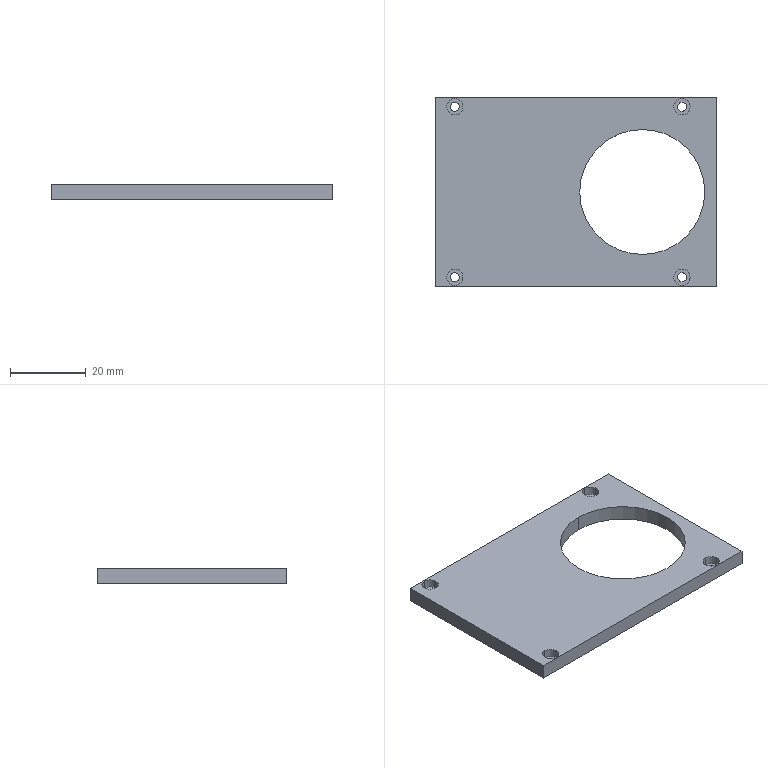CAM job | Mastercam | mm | 14 operations | part box 74 x 50 x 4
1. Facing | 24 - 80 平铣刀
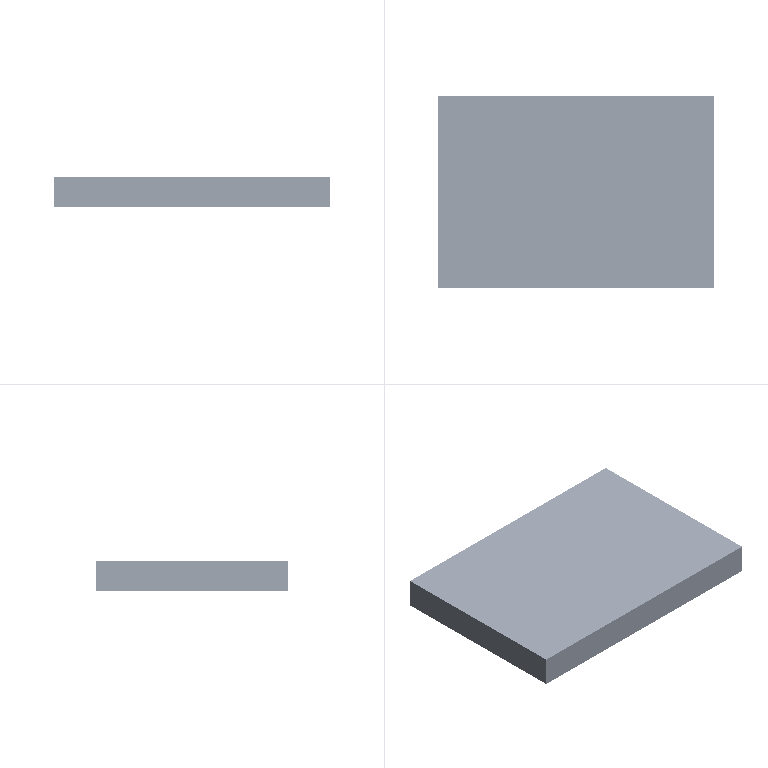2. 3D High Speed (Dynamic OptiRough) | 8 - 8C
3. Drill/Counterbore | 1 - 6 倒角刀
4. Peck Drill | 7 - 2.4 钻头
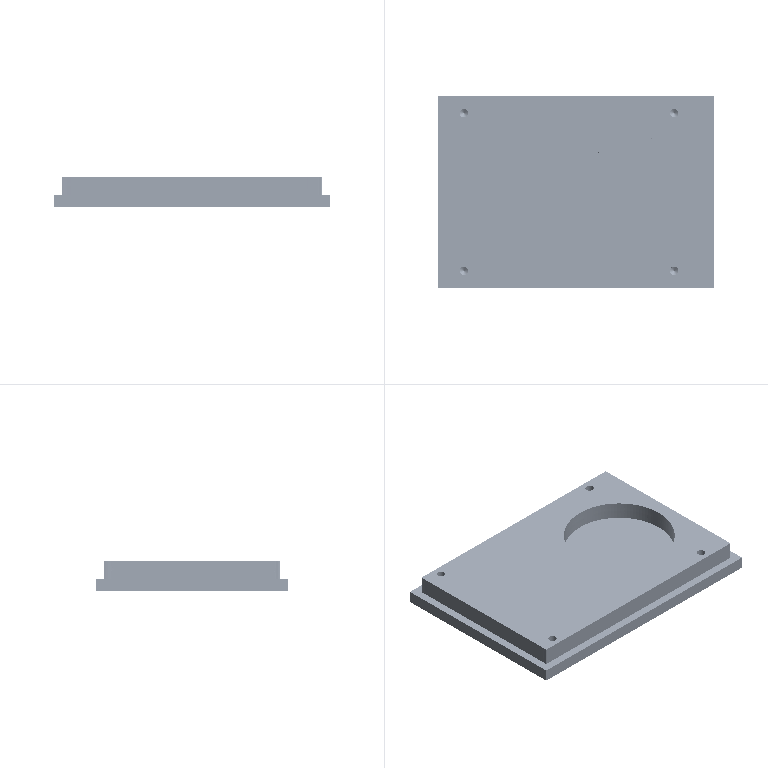5. Contour (Ramp) | 12 - 3C
6. Contour (2D) | 13 - 3J
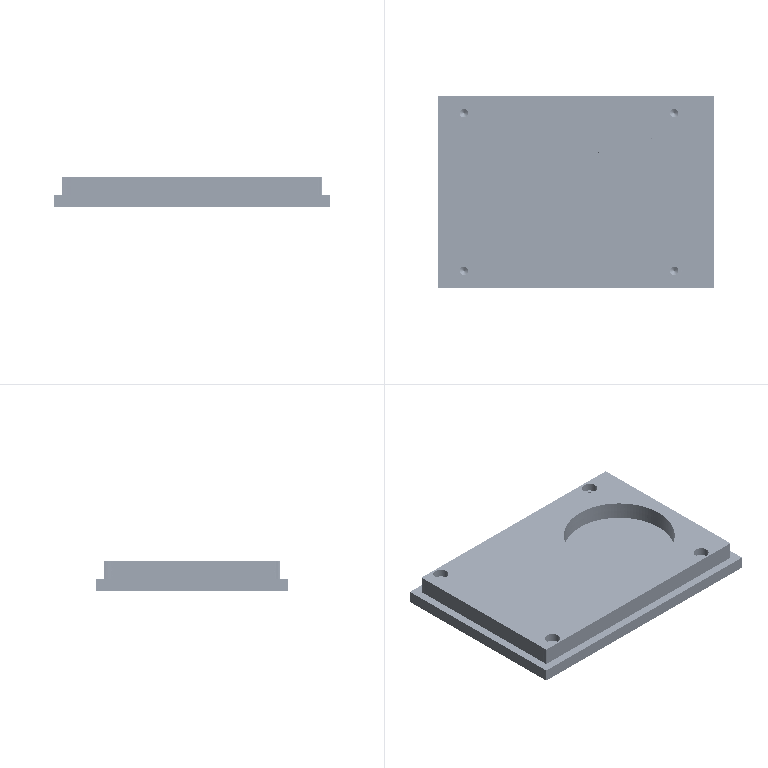7. Contour (2D) | 9 - 8J
8. Contour (2D chamfer) | 1 - 6 倒角刀
9. Facing | 24 - 80 平铣刀
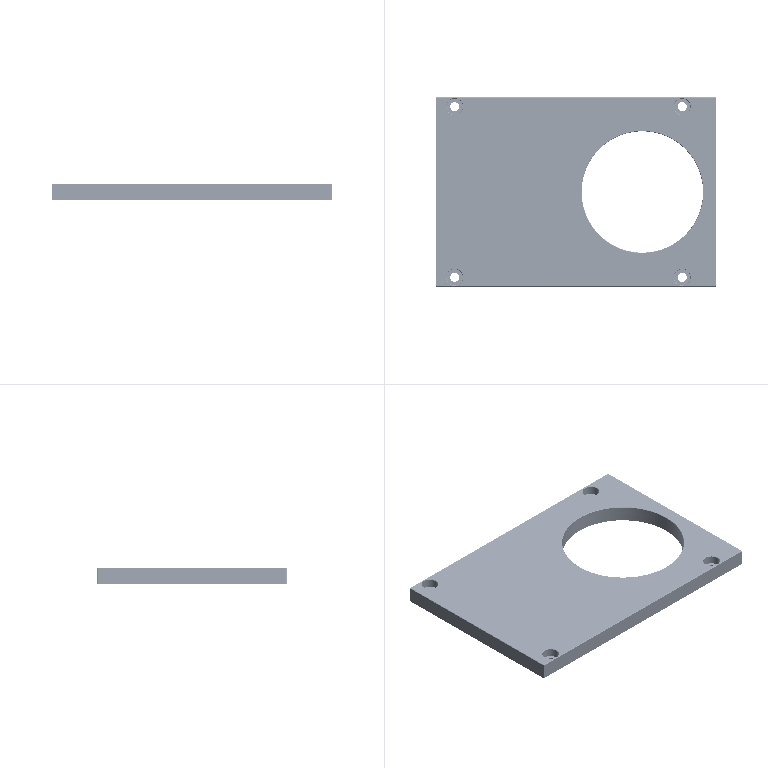10. Facing | 24 - 80 平铣刀
11. Contour (2D chamfer) | 1 - 6 倒角刀
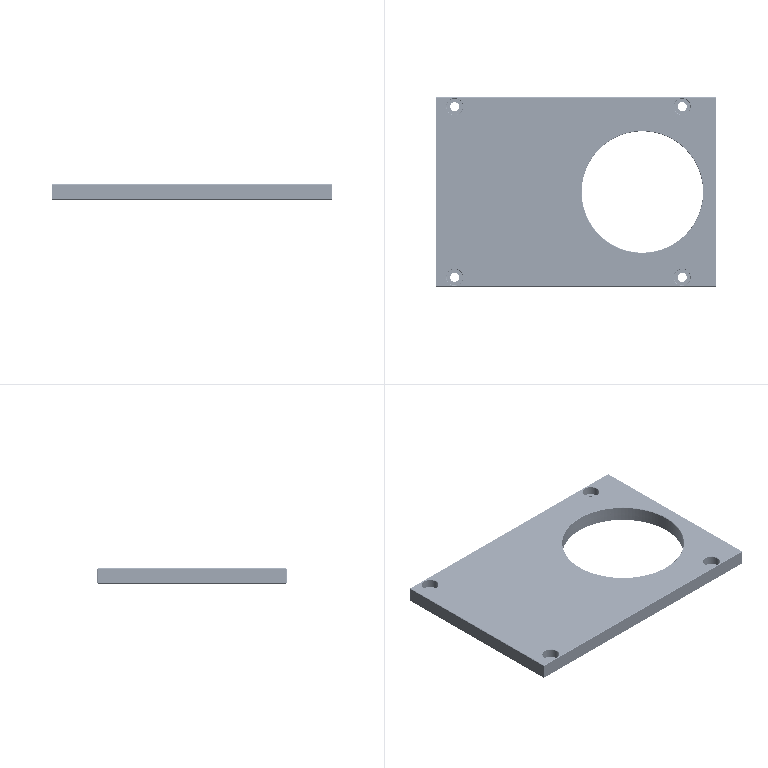12. Chamfer Drill | 1 - 6 倒角刀
13. Thread Mill | 2 - 4.75 螺纹铣刀
14. Contour (2D chamfer) | 1 - 6 倒角刀